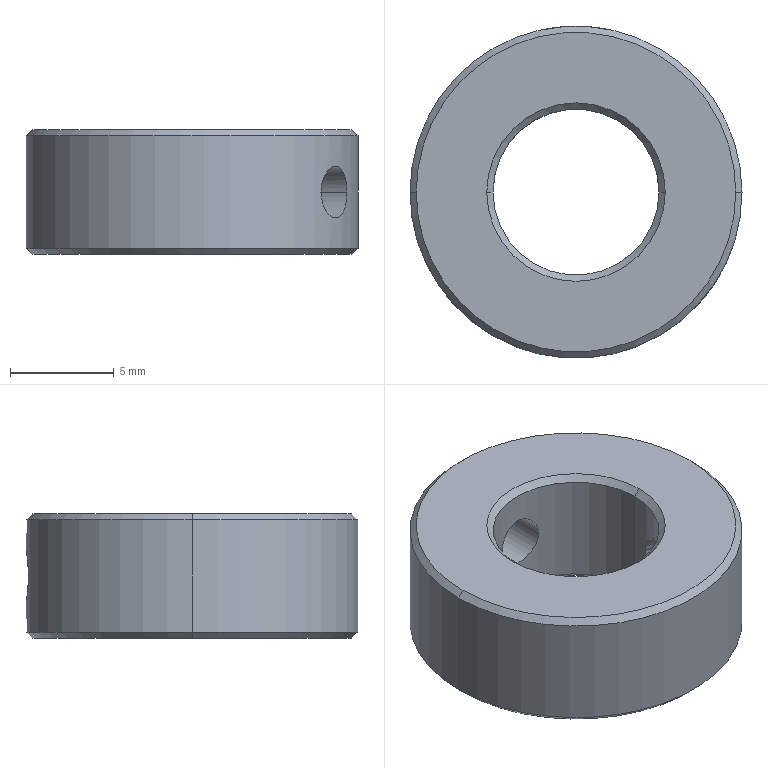Component | SolidWorks | LD101-02--Q1107-2-5 | 1 solid | 18 faces | box 16 x 16 x 6 mm | volume 858 mm3 | cylinder 8 | cone 8 | plane 2 | commonest cylinder face diameters 2.5 x4 8 x2 16 x2 | material 45
build123d program:
from build123d import *

# Parameters (mm, degrees)
SKETCH1_R           = 8
SKETCH1_R_2         = 4
BOSS_EXTRUDE1_DEPTH = 3
CHAMFER1_SIZE       = 0.3
SKETCH3_W           = 1.25
SKETCH3_H           = 8
CIRPATTERN1_COUNT   = 2
CIRPATTERN1_ANGLE   = 120


with BuildPart() as part:
    # Sketch1 → Boss-Extrude1 (new, symmetric)
    with BuildSketch(Plane.XY):
        Circle(SKETCH1_R)
        Circle(SKETCH1_R_2, mode=Mode.SUBTRACT)
    extrude(amount=BOSS_EXTRUDE1_DEPTH, both=True)

    # Chamfer1
    chamfer1_edges = [part.edges().sort_by_distance(p)[0] for p in [
        (-8, 0, -3),
        (-8, 0, 3),
        (-4, 0, -3),
        (-4, 0, 3),
    ]]
    chamfer(chamfer1_edges, length=CHAMFER1_SIZE)

    # Sketch3 → M3 Tapped Hole1 (revolve, cut)
    with BuildSketch(Plane(origin=(0, 0, 0), x_dir=(0, 0, -1), z_dir=(1, 0, 0))):
        with Locations((0.625, 4)):
            Rectangle(SKETCH3_W, SKETCH3_H)
    m3_tapped_hole1 = revolve(axis=Axis((0, -6.35, 0), (0, 1, 0)), mode=Mode.SUBTRACT)

    # CirPattern1: M3 Tapped Hole1 ×2 about axis
    cirpattern1_axis = Axis((0, 0, 3), (0, 0, -1))
    for i in range(1, CIRPATTERN1_COUNT):
        add(m3_tapped_hole1.rotate(cirpattern1_axis, i * CIRPATTERN1_ANGLE / (CIRPATTERN1_COUNT - 1)), mode=Mode.SUBTRACT)


solid = part.part

# Placed as in the assembly
solid = solid.moved(Location((79.71, -135.897, 296.257), (0, 0, 0)))
STEP:
#1=CARTESIAN_POINT('',(3.432,-5.463,11.664));
#2=VERTEX_POINT('',#1);
#3=CARTESIAN_POINT('',(3.383,-5.548,11.664));
#4=VERTEX_POINT('',#3);
#5=CARTESIAN_POINT('',(3.432,-5.463,11.664));
#6=CARTESIAN_POINT('',(3.432,-5.463,11.657));
#7=CARTESIAN_POINT('',(3.432,-5.464,11.651));
#8=CARTESIAN_POINT('',(3.43,-5.469,11.639));
#9=CARTESIAN_POINT('',(3.429,-5.472,11.633));
#10=CARTESIAN_POINT('',(3.426,-5.479,11.627));
#11=CARTESIAN_POINT('',(3.425,-5.481,11.625));
#12=CARTESIAN_POINT('',(3.422,-5.486,11.621));
#13=CARTESIAN_POINT('',(3.421,-5.488,11.619));
#14=CARTESIAN_POINT('',(3.417,-5.496,11.616));
#15=CARTESIAN_POINT('',(3.414,-5.502,11.614));
#16=CARTESIAN_POINT('',(3.408,-5.513,11.614));
#17=CARTESIAN_POINT('',(3.404,-5.519,11.616));
#18=CARTESIAN_POINT('',(3.398,-5.529,11.621));
#19=CARTESIAN_POINT('',(3.395,-5.533,11.624));
#20=CARTESIAN_POINT('',(3.389,-5.541,11.633));
#21=CARTESIAN_POINT('',(3.387,-5.544,11.639));
#22=CARTESIAN_POINT('',(3.384,-5.547,11.651));
#23=CARTESIAN_POINT('',(3.383,-5.548,11.657));
#24=CARTESIAN_POINT('',(3.383,-5.548,11.664));
#25=B_SPLINE_CURVE_WITH_KNOTS('',3,(#5,#6,#7,#8,#9,#10,#11,#12,#13,#14,#15,#16,#17,#18,#19,#20,#21,#22,#23,#24),.UNSPECIFIED.,.F.,.F.,(4,2,2,2,2,2,2,2,2,4),(0.003914,0.004403,0.004892,0.005137,0.005381,0.005871,0.00636,0.006849,0.007338,0.007827),.UNSPECIFIED.);
#26=EDGE_CURVE('',#2,#4,#25,.T.);
#27=ORIENTED_EDGE('',*,*,#26,.F.);
#28=CARTESIAN_POINT('',(3.292,-5.382,11.664));
#29=VERTEX_POINT('',#28);
#30=CARTESIAN_POINT('',(3.163,-5.308,11.664));
#31=DIRECTION('',(-0.866,0.5,0.));
#32=VECTOR('',#31,39.37);
#33=LINE('',#30,#32);
#34=EDGE_CURVE('',#2,#29,#33,.T.);
#35=ORIENTED_EDGE('',*,*,#34,.T.);
#36=CARTESIAN_POINT('',(3.243,-5.468,11.664));
#37=VERTEX_POINT('',#36);
#38=CARTESIAN_POINT('',(3.292,-5.382,11.664));
#39=CARTESIAN_POINT('',(3.292,-5.382,11.657));
#40=CARTESIAN_POINT('',(3.292,-5.384,11.651));
#41=CARTESIAN_POINT('',(3.291,-5.389,11.639));
#42=CARTESIAN_POINT('',(3.29,-5.392,11.633));
#43=CARTESIAN_POINT('',(3.287,-5.401,11.624));
#44=CARTESIAN_POINT('',(3.285,-5.407,11.621));
#45=CARTESIAN_POINT('',(3.282,-5.415,11.617));
#46=CARTESIAN_POINT('',(3.281,-5.418,11.616));
#47=CARTESIAN_POINT('',(3.278,-5.423,11.615));
#48=CARTESIAN_POINT('',(3.276,-5.426,11.614));
#49=CARTESIAN_POINT('',(3.271,-5.435,11.614));
#50=CARTESIAN_POINT('',(3.268,-5.44,11.616));
#51=CARTESIAN_POINT('',(3.261,-5.45,11.621));
#52=CARTESIAN_POINT('',(3.257,-5.454,11.624));
#53=CARTESIAN_POINT('',(3.251,-5.461,11.633));
#54=CARTESIAN_POINT('',(3.248,-5.463,11.639));
#55=CARTESIAN_POINT('',(3.244,-5.467,11.651));
#56=CARTESIAN_POINT('',(3.243,-5.468,11.657));
#57=CARTESIAN_POINT('',(3.243,-5.468,11.664));
#58=B_SPLINE_CURVE_WITH_KNOTS('',3,(#38,#39,#40,#41,#42,#43,#44,#45,#46,#47,#48,#49,#50,#51,#52,#53,#54,#55,#56,#57),.UNSPECIFIED.,.F.,.F.,(4,2,2,2,2,2,2,2,2,4),(0.003933,0.004424,0.004916,0.005407,0.005653,0.005899,0.00639,0.006882,0.007373,0.007864),.UNSPECIFIED.);
#59=EDGE_CURVE('',#29,#37,#58,.T.);
#60=ORIENTED_EDGE('',*,*,#59,.T.);
#61=CARTESIAN_POINT('',(3.114,-5.393,11.664));
#62=DIRECTION('',(-0.866,0.5,0.));
#63=VECTOR('',#62,39.37);
#64=LINE('',#61,#63);
#65=EDGE_CURVE('',#4,#37,#64,.T.);
#66=ORIENTED_EDGE('',*,*,#65,.F.);
#67=EDGE_LOOP('',(#27,#35,#60,#66));
#68=FACE_OUTER_BOUND('',#67,.T.);
#69=CARTESIAN_POINT('',(3.138,-5.35,11.664));
#70=DIRECTION('',(-0.866,0.5,0.));
#71=DIRECTION('',(-0.5,-0.866,0.));
#72=AXIS2_PLACEMENT_3D('',#69,#70,#71);
#73=CYLINDRICAL_SURFACE('',#72,0.04921);
#74=ADVANCED_FACE('',(#68),#73,.F.);
#75=CARTESIAN_POINT('',(3.138,-5.035,11.713));
#76=VERTEX_POINT('',#75);
#77=CARTESIAN_POINT('',(3.138,-5.035,11.614));
#78=VERTEX_POINT('',#77);
#79=CARTESIAN_POINT('',(3.138,-5.035,11.713));
#80=CARTESIAN_POINT('',(3.132,-5.035,11.713));
#81=CARTESIAN_POINT('',(3.125,-5.036,11.712));
#82=CARTESIAN_POINT('',(3.113,-5.036,11.707));
#83=CARTESIAN_POINT('',(3.108,-5.037,11.703));
#84=CARTESIAN_POINT('',(3.101,-5.037,11.696));
#85=CARTESIAN_POINT('',(3.099,-5.038,11.694));
#86=CARTESIAN_POINT('',(3.096,-5.038,11.688));
#87=CARTESIAN_POINT('',(3.094,-5.038,11.686));
#88=CARTESIAN_POINT('',(3.09,-5.039,11.677));
#89=CARTESIAN_POINT('',(3.089,-5.039,11.67));
#90=CARTESIAN_POINT('',(3.089,-5.039,11.657));
#91=CARTESIAN_POINT('',(3.09,-5.039,11.651));
#92=CARTESIAN_POINT('',(3.095,-5.038,11.639));
#93=CARTESIAN_POINT('',(3.099,-5.038,11.633));
#94=CARTESIAN_POINT('',(3.108,-5.037,11.624));
#95=CARTESIAN_POINT('',(3.113,-5.036,11.621));
#96=CARTESIAN_POINT('',(3.125,-5.036,11.616));
#97=CARTESIAN_POINT('',(3.132,-5.035,11.614));
#98=CARTESIAN_POINT('',(3.138,-5.035,11.614));
#99=B_SPLINE_CURVE_WITH_KNOTS('',3,(#79,#80,#81,#82,#83,#84,#85,#86,#87,#88,#89,#90,#91,#92,#93,#94,#95,#96,#97,#98),.UNSPECIFIED.,.F.,.F.,(4,2,2,2,2,2,2,2,2,4),(0.003914,0.004403,0.004892,0.005137,0.005381,0.005871,0.00636,0.006849,0.007338,0.007827),.UNSPECIFIED.);
#100=EDGE_CURVE('',#76,#78,#99,.T.);
#101=ORIENTED_EDGE('',*,*,#100,.F.);
#102=CARTESIAN_POINT('',(3.138,-5.193,11.713));
#103=VERTEX_POINT('',#102);
#104=CARTESIAN_POINT('',(3.138,-5.35,11.713));
#105=DIRECTION('',(0.,-1.,0.));
#106=VECTOR('',#105,39.37);
#107=LINE('',#104,#106);
#108=EDGE_CURVE('',#76,#103,#107,.T.);
#109=ORIENTED_EDGE('',*,*,#108,.T.);
#110=CARTESIAN_POINT('',(3.138,-5.193,11.614));
#111=VERTEX_POINT('',#110);
#112=CARTESIAN_POINT('',(3.138,-5.193,11.713));
#113=CARTESIAN_POINT('',(3.132,-5.193,11.713));
#114=CARTESIAN_POINT('',(3.125,-5.193,11.712));
#115=CARTESIAN_POINT('',(3.113,-5.195,11.707));
#116=CARTESIAN_POINT('',(3.108,-5.196,11.703));
#117=CARTESIAN_POINT('',(3.099,-5.198,11.694));
#118=CARTESIAN_POINT('',(3.095,-5.199,11.689));
#119=CARTESIAN_POINT('',(3.092,-5.2,11.68));
#120=CARTESIAN_POINT('',(3.091,-5.2,11.676));
#121=CARTESIAN_POINT('',(3.089,-5.201,11.67));
#122=CARTESIAN_POINT('',(3.089,-5.201,11.667));
#123=CARTESIAN_POINT('',(3.089,-5.201,11.657));
#124=CARTESIAN_POINT('',(3.09,-5.2,11.651));
#125=CARTESIAN_POINT('',(3.095,-5.199,11.639));
#126=CARTESIAN_POINT('',(3.099,-5.198,11.633));
#127=CARTESIAN_POINT('',(3.108,-5.196,11.624));
#128=CARTESIAN_POINT('',(3.113,-5.195,11.621));
#129=CARTESIAN_POINT('',(3.125,-5.193,11.616));
#130=CARTESIAN_POINT('',(3.132,-5.193,11.614));
#131=CARTESIAN_POINT('',(3.138,-5.193,11.614));
#132=B_SPLINE_CURVE_WITH_KNOTS('',3,(#112,#113,#114,#115,#116,#117,#118,#119,#120,#121,#122,#123,#124,#125,#126,#127,#128,#129,#130,#131),.UNSPECIFIED.,.F.,.F.,(4,2,2,2,2,2,2,2,2,4),(0.003933,0.004424,0.004916,0.005407,0.005653,0.005899,0.00639,0.006882,0.007373,0.007865),.UNSPECIFIED.);
#133=EDGE_CURVE('',#103,#111,#132,.T.);
#134=ORIENTED_EDGE('',*,*,#133,.T.);
#135=CARTESIAN_POINT('',(3.138,-5.35,11.614));
#136=DIRECTION('',(0.,-1.,0.));
#137=VECTOR('',#136,39.37);
#138=LINE('',#135,#137);
#139=EDGE_CURVE('',#78,#111,#138,.T.);
#140=ORIENTED_EDGE('',*,*,#139,.F.);
#141=EDGE_LOOP('',(#101,#109,#134,#140));
#142=FACE_OUTER_BOUND('',#141,.T.);
#143=CARTESIAN_POINT('',(3.138,-5.35,11.664));
#144=DIRECTION('',(0.,-1.,0.));
#145=DIRECTION('',(0.,0.,-1.));
#146=AXIS2_PLACEMENT_3D('',#143,#144,#145);
#147=CYLINDRICAL_SURFACE('',#146,0.04921);
#148=ADVANCED_FACE('',(#142),#147,.F.);
#149=CARTESIAN_POINT('',(3.441,-5.35,11.782));
#150=VERTEX_POINT('',#149);
#151=CARTESIAN_POINT('',(2.835,-5.35,11.782));
#152=VERTEX_POINT('',#151);
#153=CARTESIAN_POINT('',(3.138,-5.35,11.782));
#154=DIRECTION('',(0.,0.,1.));
#155=DIRECTION('',(1.,0.,0.));
#156=AXIS2_PLACEMENT_3D('',#153,#154,#155);
#157=CIRCLE('',#156,0.3031);
#158=EDGE_CURVE('',#150,#152,#157,.T.);
#159=ORIENTED_EDGE('',*,*,#158,.F.);
#160=CARTESIAN_POINT('',(3.453,-5.35,11.77));
#161=VERTEX_POINT('',#160);
#162=CARTESIAN_POINT('',(3.441,-5.35,11.782));
#163=DIRECTION('',(0.7071,0.,-0.7071));
#164=VECTOR('',#163,39.37);
#165=LINE('',#162,#164);
#166=EDGE_CURVE('',#150,#161,#165,.T.);
#167=ORIENTED_EDGE('',*,*,#166,.T.);
#168=CARTESIAN_POINT('',(2.823,-5.35,11.77));
#169=VERTEX_POINT('',#168);
#170=CARTESIAN_POINT('',(3.138,-5.35,11.77));
#171=DIRECTION('',(0.,0.,-1.));
#172=DIRECTION('',(1.,0.,0.));
#173=AXIS2_PLACEMENT_3D('',#170,#171,#172);
#174=CIRCLE('',#173,0.315);
#175=EDGE_CURVE('',#169,#161,#174,.T.);
#176=ORIENTED_EDGE('',*,*,#175,.F.);
#177=CARTESIAN_POINT('',(2.835,-5.35,11.782));
#178=DIRECTION('',(-0.7071,0.,-0.7071));
#179=VECTOR('',#178,39.37);
#180=LINE('',#177,#179);
#181=EDGE_CURVE('',#152,#169,#180,.T.);
#182=ORIENTED_EDGE('',*,*,#181,.F.);
#183=EDGE_LOOP('',(#159,#167,#176,#182));
#184=FACE_OUTER_BOUND('',#183,.T.);
#185=CARTESIAN_POINT('',(3.138,-5.35,11.782));
#186=DIRECTION('',(0.,0.,-1.));
#187=DIRECTION('',(-1.,0.,0.));
#188=AXIS2_PLACEMENT_3D('',#185,#186,#187);
#189=CONICAL_SURFACE('',#188,0.3031,0.7854);
#190=ADVANCED_FACE('',(#184),#189,.T.);
#191=CARTESIAN_POINT('',(2.981,-5.35,11.77));
#192=VERTEX_POINT('',#191);
#193=CARTESIAN_POINT('',(3.296,-5.35,11.77));
#194=VERTEX_POINT('',#193);
#195=CARTESIAN_POINT('',(3.138,-5.35,11.77));
#196=DIRECTION('',(0.,0.,1.));
#197=DIRECTION('',(1.,0.,0.));
#198=AXIS2_PLACEMENT_3D('',#195,#196,#197);
#199=CIRCLE('',#198,0.1575);
#200=EDGE_CURVE('',#192,#194,#199,.T.);
#201=ORIENTED_EDGE('',*,*,#200,.F.);
#202=CARTESIAN_POINT('',(2.969,-5.35,11.782));
#203=VERTEX_POINT('',#202);
#204=CARTESIAN_POINT('',(2.981,-5.35,11.77));
#205=DIRECTION('',(-0.7071,0.,0.7071));
#206=VECTOR('',#205,39.37);
#207=LINE('',#204,#206);
#208=EDGE_CURVE('',#192,#203,#207,.T.);
#209=ORIENTED_EDGE('',*,*,#208,.T.);
#210=CARTESIAN_POINT('',(3.307,-5.35,11.782));
#211=VERTEX_POINT('',#210);
#212=CARTESIAN_POINT('',(3.138,-5.35,11.782));
#213=DIRECTION('',(0.,0.,-1.));
#214=DIRECTION('',(1.,0.,0.));
#215=AXIS2_PLACEMENT_3D('',#212,#213,#214);
#216=CIRCLE('',#215,0.1693);
#217=EDGE_CURVE('',#211,#203,#216,.T.);
#218=ORIENTED_EDGE('',*,*,#217,.F.);
#219=CARTESIAN_POINT('',(3.296,-5.35,11.77));
#220=DIRECTION('',(0.7071,0.,0.7071));
#221=VECTOR('',#220,39.37);
#222=LINE('',#219,#221);
#223=EDGE_CURVE('',#194,#211,#222,.T.);
#224=ORIENTED_EDGE('',*,*,#223,.F.);
#225=EDGE_LOOP('',(#201,#209,#218,#224));
#226=FACE_OUTER_BOUND('',#225,.T.);
#227=CARTESIAN_POINT('',(3.138,-5.35,11.77));
#228=DIRECTION('',(0.,0.,1.));
#229=DIRECTION('',(1.,0.,0.));
#230=AXIS2_PLACEMENT_3D('',#227,#228,#229);
#231=CONICAL_SURFACE('',#230,0.1575,0.7854);
#232=ADVANCED_FACE('',(#226),#231,.F.);
#233=CARTESIAN_POINT('',(2.835,-5.35,11.546));
#234=VERTEX_POINT('',#233);
#235=CARTESIAN_POINT('',(3.441,-5.35,11.546));
#236=VERTEX_POINT('',#235);
#237=CARTESIAN_POINT('',(3.138,-5.35,11.546));
#238=DIRECTION('',(0.,0.,-1.));
#239=DIRECTION('',(1.,0.,0.));
#240=AXIS2_PLACEMENT_3D('',#237,#238,#239);
#241=CIRCLE('',#240,0.3031);
#242=EDGE_CURVE('',#234,#236,#241,.T.);
#243=ORIENTED_EDGE('',*,*,#242,.F.);
#244=CARTESIAN_POINT('',(2.823,-5.35,11.557));
#245=VERTEX_POINT('',#244);
#246=CARTESIAN_POINT('',(2.823,-5.35,11.557));
#247=DIRECTION('',(-0.7071,0.,0.7071));
#248=VECTOR('',#247,39.37);
#249=LINE('',#246,#248);
#250=EDGE_CURVE('',#234,#245,#249,.T.);
#251=ORIENTED_EDGE('',*,*,#250,.T.);
#252=CARTESIAN_POINT('',(3.453,-5.35,11.557));
#253=VERTEX_POINT('',#252);
#254=CARTESIAN_POINT('',(3.138,-5.35,11.557));
#255=DIRECTION('',(0.,0.,1.));
#256=DIRECTION('',(1.,0.,0.));
#257=AXIS2_PLACEMENT_3D('',#254,#255,#256);
#258=CIRCLE('',#257,0.315);
#259=EDGE_CURVE('',#253,#245,#258,.T.);
#260=ORIENTED_EDGE('',*,*,#259,.F.);
#261=CARTESIAN_POINT('',(3.453,-5.35,11.557));
#262=DIRECTION('',(0.7071,0.,0.7071));
#263=VECTOR('',#262,39.37);
#264=LINE('',#261,#263);
#265=EDGE_CURVE('',#236,#253,#264,.T.);
#266=ORIENTED_EDGE('',*,*,#265,.F.);
#267=EDGE_LOOP('',(#243,#251,#260,#266));
#268=FACE_OUTER_BOUND('',#267,.T.);
#269=CARTESIAN_POINT('',(3.138,-5.35,11.557));
#270=DIRECTION('',(0.,0.,1.));
#271=DIRECTION('',(1.,0.,0.));
#272=AXIS2_PLACEMENT_3D('',#269,#270,#271);
#273=CONICAL_SURFACE('',#272,0.315,0.7854);
#274=ADVANCED_FACE('',(#268),#273,.T.);
#275=CARTESIAN_POINT('',(3.296,-5.35,11.557));
#276=VERTEX_POINT('',#275);
#277=CARTESIAN_POINT('',(2.981,-5.35,11.557));
#278=VERTEX_POINT('',#277);
#279=CARTESIAN_POINT('',(3.138,-5.35,11.557));
#280=DIRECTION('',(0.,0.,-1.));
#281=DIRECTION('',(1.,0.,0.));
#282=AXIS2_PLACEMENT_3D('',#279,#280,#281);
#283=CIRCLE('',#282,0.1575);
#284=EDGE_CURVE('',#276,#278,#283,.T.);
#285=ORIENTED_EDGE('',*,*,#284,.F.);
#286=CARTESIAN_POINT('',(3.307,-5.35,11.546));
#287=VERTEX_POINT('',#286);
#288=CARTESIAN_POINT('',(3.307,-5.35,11.546));
#289=DIRECTION('',(0.7071,0.,-0.7071));
#290=VECTOR('',#289,39.37);
#291=LINE('',#288,#290);
#292=EDGE_CURVE('',#276,#287,#291,.T.);
#293=ORIENTED_EDGE('',*,*,#292,.T.);
#294=CARTESIAN_POINT('',(2.969,-5.35,11.546));
#295=VERTEX_POINT('',#294);
#296=CARTESIAN_POINT('',(3.138,-5.35,11.546));
#297=DIRECTION('',(0.,0.,1.));
#298=DIRECTION('',(1.,0.,0.));
#299=AXIS2_PLACEMENT_3D('',#296,#297,#298);
#300=CIRCLE('',#299,0.1693);
#301=EDGE_CURVE('',#295,#287,#300,.T.);
#302=ORIENTED_EDGE('',*,*,#301,.F.);
#303=CARTESIAN_POINT('',(2.969,-5.35,11.546));
#304=DIRECTION('',(-0.7071,0.,-0.7071));
#305=VECTOR('',#304,39.37);
#306=LINE('',#303,#305);
#307=EDGE_CURVE('',#278,#295,#306,.T.);
#308=ORIENTED_EDGE('',*,*,#307,.F.);
#309=EDGE_LOOP('',(#285,#293,#302,#308));
#310=FACE_OUTER_BOUND('',#309,.T.);
#311=CARTESIAN_POINT('',(3.138,-5.35,11.546));
#312=DIRECTION('',(0.,0.,-1.));
#313=DIRECTION('',(-1.,0.,0.));
#314=AXIS2_PLACEMENT_3D('',#311,#312,#313);
#315=CONICAL_SURFACE('',#314,0.1693,0.7854);
#316=ADVANCED_FACE('',(#310),#315,.F.);
#317=CARTESIAN_POINT('',(3.243,-5.468,11.664));
#318=CARTESIAN_POINT('',(3.243,-5.468,11.67));
#319=CARTESIAN_POINT('',(3.244,-5.467,11.677));
#320=CARTESIAN_POINT('',(3.248,-5.463,11.689));
#321=CARTESIAN_POINT('',(3.251,-5.461,11.694));
#322=CARTESIAN_POINT('',(3.257,-5.454,11.703));
#323=CARTESIAN_POINT('',(3.261,-5.45,11.707));
#324=CARTESIAN_POINT('',(3.268,-5.44,11.712));
#325=CARTESIAN_POINT('',(3.271,-5.435,11.713));
#326=CARTESIAN_POINT('',(3.276,-5.426,11.713));
#327=CARTESIAN_POINT('',(3.278,-5.423,11.713));
#328=CARTESIAN_POINT('',(3.281,-5.418,11.711));
#329=CARTESIAN_POINT('',(3.282,-5.415,11.71));
#330=CARTESIAN_POINT('',(3.285,-5.407,11.707));
#331=CARTESIAN_POINT('',(3.287,-5.401,11.703));
#332=CARTESIAN_POINT('',(3.289,-5.395,11.696));
#333=CARTESIAN_POINT('',(3.29,-5.393,11.694));
#334=CARTESIAN_POINT('',(3.291,-5.389,11.688));
#335=CARTESIAN_POINT('',(3.291,-5.388,11.685));
#336=CARTESIAN_POINT('',(3.292,-5.384,11.677));
#337=CARTESIAN_POINT('',(3.292,-5.382,11.67));
#338=CARTESIAN_POINT('',(3.292,-5.382,11.664));
#339=B_SPLINE_CURVE_WITH_KNOTS('',3,(#317,#318,#319,#320,#321,#322,#323,#324,#325,#326,#327,#328,#329,#330,#331,#332,#333,#334,#335,#336,#337,#338),.UNSPECIFIED.,.F.,.F.,(4,2,2,2,2,2,2,2,2,2,4),(0.,0.0004916,0.0009832,0.001475,0.001966,0.002212,0.002458,0.00295,0.003195,0.003441,0.003933),.UNSPECIFIED.);
#340=EDGE_CURVE('',#37,#29,#339,.T.);
#341=ORIENTED_EDGE('',*,*,#340,.F.);
#342=ORIENTED_EDGE('',*,*,#59,.F.);
#343=EDGE_LOOP('',(#341,#342));
#344=FACE_BOUND('',#343,.T.);
#345=ORIENTED_EDGE('',*,*,#200,.T.);
#346=CARTESIAN_POINT('',(3.296,-5.35,11.782));
#347=DIRECTION('',(0.,0.,-1.));
#348=VECTOR('',#347,39.37);
#349=LINE('',#346,#348);
#350=EDGE_CURVE('',#194,#276,#349,.T.);
#351=ORIENTED_EDGE('',*,*,#350,.T.);
#352=ORIENTED_EDGE('',*,*,#284,.T.);
#353=CARTESIAN_POINT('',(2.981,-5.35,11.782));
#354=DIRECTION('',(0.,0.,-1.));
#355=VECTOR('',#354,39.37);
#356=LINE('',#353,#355);
#357=EDGE_CURVE('',#192,#278,#356,.T.);
#358=ORIENTED_EDGE('',*,*,#357,.F.);
#359=EDGE_LOOP('',(#345,#351,#352,#358));
#360=FACE_OUTER_BOUND('',#359,.T.);
#361=CARTESIAN_POINT('',(3.138,-5.35,11.782));
#362=DIRECTION('',(0.,0.,-1.));
#363=DIRECTION('',(-1.,0.,0.));
#364=AXIS2_PLACEMENT_3D('',#361,#362,#363);
#365=CYLINDRICAL_SURFACE('',#364,0.1575);
#366=ADVANCED_FACE('',(#344,#360),#365,.F.);
#367=CARTESIAN_POINT('',(3.138,-5.035,11.614));
#368=CARTESIAN_POINT('',(3.145,-5.035,11.614));
#369=CARTESIAN_POINT('',(3.151,-5.036,11.616));
#370=CARTESIAN_POINT('',(3.163,-5.036,11.621));
#371=CARTESIAN_POINT('',(3.168,-5.037,11.624));
#372=CARTESIAN_POINT('',(3.178,-5.038,11.633));
#373=CARTESIAN_POINT('',(3.181,-5.038,11.639));
#374=CARTESIAN_POINT('',(3.186,-5.039,11.651));
#375=CARTESIAN_POINT('',(3.187,-5.039,11.657));
#376=CARTESIAN_POINT('',(3.187,-5.039,11.667));
#377=CARTESIAN_POINT('',(3.187,-5.039,11.67));
#378=CARTESIAN_POINT('',(3.186,-5.039,11.676));
#379=CARTESIAN_POINT('',(3.185,-5.039,11.679));
#380=CARTESIAN_POINT('',(3.181,-5.038,11.688));
#381=CARTESIAN_POINT('',(3.178,-5.038,11.694));
#382=CARTESIAN_POINT('',(3.168,-5.037,11.703));
#383=CARTESIAN_POINT('',(3.163,-5.036,11.707));
#384=CARTESIAN_POINT('',(3.154,-5.036,11.71));
#385=CARTESIAN_POINT('',(3.151,-5.036,11.711));
#386=CARTESIAN_POINT('',(3.145,-5.035,11.713));
#387=CARTESIAN_POINT('',(3.141,-5.035,11.713));
#388=CARTESIAN_POINT('',(3.138,-5.035,11.713));
#389=B_SPLINE_CURVE_WITH_KNOTS('',3,(#367,#368,#369,#370,#371,#372,#373,#374,#375,#376,#377,#378,#379,#380,#381,#382,#383,#384,#385,#386,#387,#388),.UNSPECIFIED.,.F.,.F.,(4,2,2,2,2,2,2,2,2,2,4),(0.,0.0004893,0.0009785,0.001468,0.001957,0.002202,0.002446,0.002936,0.003425,0.003669,0.003914),.UNSPECIFIED.);
#390=EDGE_CURVE('',#78,#76,#389,.T.);
#391=ORIENTED_EDGE('',*,*,#390,.T.);
#392=ORIENTED_EDGE('',*,*,#100,.T.);
#393=EDGE_LOOP('',(#391,#392));
#394=FACE_BOUND('',#393,.T.);
#395=ORIENTED_EDGE('',*,*,#175,.T.);
#396=CARTESIAN_POINT('',(3.453,-5.35,11.782));
#397=DIRECTION('',(0.,0.,-1.));
#398=VECTOR('',#397,39.37);
#399=LINE('',#396,#398);
#400=EDGE_CURVE('',#161,#253,#399,.T.);
#401=ORIENTED_EDGE('',*,*,#400,.T.);
#402=ORIENTED_EDGE('',*,*,#259,.T.);
#403=CARTESIAN_POINT('',(2.823,-5.35,11.782));
#404=DIRECTION('',(0.,0.,-1.));
#405=VECTOR('',#404,39.37);
#406=LINE('',#403,#405);
#407=EDGE_CURVE('',#169,#245,#406,.T.);
#408=ORIENTED_EDGE('',*,*,#407,.F.);
#409=EDGE_LOOP('',(#395,#401,#402,#408));
#410=FACE_OUTER_BOUND('',#409,.T.);
#411=CARTESIAN_POINT('',(3.138,-5.35,11.782));
#412=DIRECTION('',(0.,0.,-1.));
#413=DIRECTION('',(-1.,0.,0.));
#414=AXIS2_PLACEMENT_3D('',#411,#412,#413);
#415=CYLINDRICAL_SURFACE('',#414,0.315);
#416=ADVANCED_FACE('',(#394,#410),#415,.T.);
#417=ORIENTED_EDGE('',*,*,#217,.T.);
#418=CARTESIAN_POINT('',(3.138,-5.35,11.782));
#419=DIRECTION('',(0.,0.,-1.));
#420=DIRECTION('',(1.,0.,0.));
#421=AXIS2_PLACEMENT_3D('',#418,#419,#420);
#422=CIRCLE('',#421,0.1693);
#423=EDGE_CURVE('',#203,#211,#422,.T.);
#424=ORIENTED_EDGE('',*,*,#423,.T.);
#425=EDGE_LOOP('',(#417,#424));
#426=FACE_BOUND('',#425,.T.);
#427=CARTESIAN_POINT('',(3.138,-5.35,11.782));
#428=DIRECTION('',(0.,0.,1.));
#429=DIRECTION('',(1.,0.,0.));
#430=AXIS2_PLACEMENT_3D('',#427,#428,#429);
#431=CIRCLE('',#430,0.3031);
#432=EDGE_CURVE('',#152,#150,#431,.T.);
#433=ORIENTED_EDGE('',*,*,#432,.T.);
#434=ORIENTED_EDGE('',*,*,#158,.T.);
#435=EDGE_LOOP('',(#433,#434));
#436=FACE_OUTER_BOUND('',#435,.T.);
#437=CARTESIAN_POINT('',(3.138,-5.35,11.782));
#438=DIRECTION('',(0.,0.,1.));
#439=DIRECTION('',(1.,0.,0.));
#440=AXIS2_PLACEMENT_3D('',#437,#438,#439);
#441=PLANE('',#440);
#442=ADVANCED_FACE('',(#426,#436),#441,.T.);
#443=ORIENTED_EDGE('',*,*,#301,.T.);
#444=CARTESIAN_POINT('',(3.138,-5.35,11.546));
#445=DIRECTION('',(0.,0.,1.));
#446=DIRECTION('',(1.,0.,0.));
#447=AXIS2_PLACEMENT_3D('',#444,#445,#446);
#448=CIRCLE('',#447,0.1693);
#449=EDGE_CURVE('',#287,#295,#448,.T.);
#450=ORIENTED_EDGE('',*,*,#449,.T.);
#451=EDGE_LOOP('',(#443,#450));
#452=FACE_BOUND('',#451,.T.);
#453=CARTESIAN_POINT('',(3.138,-5.35,11.546));
#454=DIRECTION('',(0.,0.,-1.));
#455=DIRECTION('',(1.,0.,0.));
#456=AXIS2_PLACEMENT_3D('',#453,#454,#455);
#457=CIRCLE('',#456,0.3031);
#458=EDGE_CURVE('',#236,#234,#457,.T.);
#459=ORIENTED_EDGE('',*,*,#458,.T.);
#460=ORIENTED_EDGE('',*,*,#242,.T.);
#461=EDGE_LOOP('',(#459,#460));
#462=FACE_OUTER_BOUND('',#461,.T.);
#463=CARTESIAN_POINT('',(3.138,-5.35,11.546));
#464=DIRECTION('',(0.,0.,1.));
#465=DIRECTION('',(1.,0.,0.));
#466=AXIS2_PLACEMENT_3D('',#463,#464,#465);
#467=PLANE('',#466);
#468=ADVANCED_FACE('',(#452,#462),#467,.F.);
#469=ORIENTED_EDGE('',*,*,#400,.F.);
#470=CARTESIAN_POINT('',(3.138,-5.35,11.77));
#471=DIRECTION('',(0.,0.,-1.));
#472=DIRECTION('',(1.,0.,0.));
#473=AXIS2_PLACEMENT_3D('',#470,#471,#472);
#474=CIRCLE('',#473,0.315);
#475=EDGE_CURVE('',#161,#169,#474,.T.);
#476=ORIENTED_EDGE('',*,*,#475,.T.);
#477=ORIENTED_EDGE('',*,*,#407,.T.);
#478=CARTESIAN_POINT('',(3.138,-5.35,11.557));
#479=DIRECTION('',(0.,0.,1.));
#480=DIRECTION('',(1.,0.,0.));
#481=AXIS2_PLACEMENT_3D('',#478,#479,#480);
#482=CIRCLE('',#481,0.315);
#483=EDGE_CURVE('',#245,#253,#482,.T.);
#484=ORIENTED_EDGE('',*,*,#483,.T.);
#485=EDGE_LOOP('',(#469,#476,#477,#484));
#486=FACE_OUTER_BOUND('',#485,.T.);
#487=CARTESIAN_POINT('',(3.383,-5.548,11.664));
#488=CARTESIAN_POINT('',(3.383,-5.548,11.67));
#489=CARTESIAN_POINT('',(3.384,-5.547,11.677));
#490=CARTESIAN_POINT('',(3.387,-5.544,11.688));
#491=CARTESIAN_POINT('',(3.389,-5.541,11.694));
#492=CARTESIAN_POINT('',(3.395,-5.533,11.703));
#493=CARTESIAN_POINT('',(3.398,-5.529,11.707));
#494=CARTESIAN_POINT('',(3.404,-5.519,11.712));
#495=CARTESIAN_POINT('',(3.408,-5.513,11.713));
#496=CARTESIAN_POINT('',(3.413,-5.505,11.713));
#497=CARTESIAN_POINT('',(3.414,-5.502,11.713));
#498=CARTESIAN_POINT('',(3.417,-5.497,11.711));
#499=CARTESIAN_POINT('',(3.419,-5.494,11.71));
#500=CARTESIAN_POINT('',(3.423,-5.486,11.707));
#501=CARTESIAN_POINT('',(3.425,-5.481,11.703));
#502=CARTESIAN_POINT('',(3.429,-5.472,11.694));
#503=CARTESIAN_POINT('',(3.43,-5.469,11.688));
#504=CARTESIAN_POINT('',(3.431,-5.466,11.68));
#505=CARTESIAN_POINT('',(3.432,-5.465,11.676));
#506=CARTESIAN_POINT('',(3.432,-5.464,11.67));
#507=CARTESIAN_POINT('',(3.432,-5.463,11.667));
#508=CARTESIAN_POINT('',(3.432,-5.463,11.664));
#509=B_SPLINE_CURVE_WITH_KNOTS('',3,(#487,#488,#489,#490,#491,#492,#493,#494,#495,#496,#497,#498,#499,#500,#501,#502,#503,#504,#505,#506,#507,#508),.UNSPECIFIED.,.F.,.F.,(4,2,2,2,2,2,2,2,2,2,4),(0.,0.0004893,0.0009785,0.001468,0.001957,0.002202,0.002446,0.002936,0.003425,0.003669,0.003914),.UNSPECIFIED.);
#510=EDGE_CURVE('',#4,#2,#509,.T.);
#511=ORIENTED_EDGE('',*,*,#510,.T.);
#512=ORIENTED_EDGE('',*,*,#26,.T.);
#513=EDGE_LOOP('',(#511,#512));
#514=FACE_BOUND('',#513,.T.);
#515=CARTESIAN_POINT('',(3.138,-5.35,11.782));
#516=DIRECTION('',(0.,0.,-1.));
#517=DIRECTION('',(-1.,0.,0.));
#518=AXIS2_PLACEMENT_3D('',#515,#516,#517);
#519=CYLINDRICAL_SURFACE('',#518,0.315);
#520=ADVANCED_FACE('',(#486,#514),#519,.T.);
#521=ORIENTED_EDGE('',*,*,#350,.F.);
#522=CARTESIAN_POINT('',(3.138,-5.35,11.77));
#523=DIRECTION('',(0.,0.,1.));
#524=DIRECTION('',(1.,0.,0.));
#525=AXIS2_PLACEMENT_3D('',#522,#523,#524);
#526=CIRCLE('',#525,0.1575);
#527=EDGE_CURVE('',#194,#192,#526,.T.);
#528=ORIENTED_EDGE('',*,*,#527,.T.);
#529=ORIENTED_EDGE('',*,*,#357,.T.);
#530=CARTESIAN_POINT('',(3.138,-5.35,11.557));
#531=DIRECTION('',(0.,0.,-1.));
#532=DIRECTION('',(1.,0.,0.));
#533=AXIS2_PLACEMENT_3D('',#530,#531,#532);
#534=CIRCLE('',#533,0.1575);
#535=EDGE_CURVE('',#278,#276,#534,.T.);
#536=ORIENTED_EDGE('',*,*,#535,.T.);
#537=EDGE_LOOP('',(#521,#528,#529,#536));
#538=FACE_OUTER_BOUND('',#537,.T.);
#539=CARTESIAN_POINT('',(3.138,-5.193,11.614));
#540=CARTESIAN_POINT('',(3.145,-5.193,11.614));
#541=CARTESIAN_POINT('',(3.151,-5.193,11.616));
#542=CARTESIAN_POINT('',(3.163,-5.195,11.621));
#543=CARTESIAN_POINT('',(3.169,-5.196,11.624));
#544=CARTESIAN_POINT('',(3.178,-5.198,11.633));
#545=CARTESIAN_POINT('',(3.181,-5.199,11.639));
#546=CARTESIAN_POINT('',(3.186,-5.2,11.651));
#547=CARTESIAN_POINT('',(3.187,-5.201,11.657));
#548=CARTESIAN_POINT('',(3.187,-5.201,11.667));
#549=CARTESIAN_POINT('',(3.187,-5.201,11.67));
#550=CARTESIAN_POINT('',(3.186,-5.2,11.676));
#551=CARTESIAN_POINT('',(3.185,-5.2,11.68));
#552=CARTESIAN_POINT('',(3.181,-5.199,11.689));
#553=CARTESIAN_POINT('',(3.178,-5.198,11.694));
#554=CARTESIAN_POINT('',(3.171,-5.196,11.701));
#555=CARTESIAN_POINT('',(3.168,-5.196,11.703));
#556=CARTESIAN_POINT('',(3.163,-5.195,11.706));
#557=CARTESIAN_POINT('',(3.16,-5.194,11.708));
#558=CARTESIAN_POINT('',(3.151,-5.193,11.712));
#559=CARTESIAN_POINT('',(3.145,-5.193,11.713));
#560=CARTESIAN_POINT('',(3.138,-5.193,11.713));
#561=B_SPLINE_CURVE_WITH_KNOTS('',3,(#539,#540,#541,#542,#543,#544,#545,#546,#547,#548,#549,#550,#551,#552,#553,#554,#555,#556,#557,#558,#559,#560),.UNSPECIFIED.,.F.,.F.,(4,2,2,2,2,2,2,2,2,2,4),(0.,0.0004916,0.0009832,0.001475,0.001966,0.002212,0.002458,0.00295,0.003195,0.003441,0.003933),.UNSPECIFIED.);
#562=EDGE_CURVE('',#111,#103,#561,.T.);
#563=ORIENTED_EDGE('',*,*,#562,.F.);
#564=ORIENTED_EDGE('',*,*,#133,.F.);
#565=EDGE_LOOP('',(#563,#564));
#566=FACE_BOUND('',#565,.T.);
#567=CARTESIAN_POINT('',(3.138,-5.35,11.782));
#568=DIRECTION('',(0.,0.,-1.));
#569=DIRECTION('',(-1.,0.,0.));
#570=AXIS2_PLACEMENT_3D('',#567,#568,#569);
#571=CYLINDRICAL_SURFACE('',#570,0.1575);
#572=ADVANCED_FACE('',(#538,#566),#571,.F.);
#573=ORIENTED_EDGE('',*,*,#292,.F.);
#574=ORIENTED_EDGE('',*,*,#535,.F.);
#575=ORIENTED_EDGE('',*,*,#307,.T.);
#576=ORIENTED_EDGE('',*,*,#449,.F.);
#577=EDGE_LOOP('',(#573,#574,#575,#576));
#578=FACE_OUTER_BOUND('',#577,.T.);
#579=CARTESIAN_POINT('',(3.138,-5.35,11.546));
#580=DIRECTION('',(0.,0.,-1.));
#581=DIRECTION('',(-1.,0.,0.));
#582=AXIS2_PLACEMENT_3D('',#579,#580,#581);
#583=CONICAL_SURFACE('',#582,0.1693,0.7854);
#584=ADVANCED_FACE('',(#578),#583,.F.);
#585=ORIENTED_EDGE('',*,*,#250,.F.);
#586=ORIENTED_EDGE('',*,*,#458,.F.);
#587=ORIENTED_EDGE('',*,*,#265,.T.);
#588=ORIENTED_EDGE('',*,*,#483,.F.);
#589=EDGE_LOOP('',(#585,#586,#587,#588));
#590=FACE_OUTER_BOUND('',#589,.T.);
#591=CARTESIAN_POINT('',(3.138,-5.35,11.557));
#592=DIRECTION('',(0.,0.,1.));
#593=DIRECTION('',(1.,0.,0.));
#594=AXIS2_PLACEMENT_3D('',#591,#592,#593);
#595=CONICAL_SURFACE('',#594,0.315,0.7854);
#596=ADVANCED_FACE('',(#590),#595,.T.);
#597=ORIENTED_EDGE('',*,*,#208,.F.);
#598=ORIENTED_EDGE('',*,*,#527,.F.);
#599=ORIENTED_EDGE('',*,*,#223,.T.);
#600=ORIENTED_EDGE('',*,*,#423,.F.);
#601=EDGE_LOOP('',(#597,#598,#599,#600));
#602=FACE_OUTER_BOUND('',#601,.T.);
#603=CARTESIAN_POINT('',(3.138,-5.35,11.77));
#604=DIRECTION('',(0.,0.,1.));
#605=DIRECTION('',(1.,0.,0.));
#606=AXIS2_PLACEMENT_3D('',#603,#604,#605);
#607=CONICAL_SURFACE('',#606,0.1575,0.7854);
#608=ADVANCED_FACE('',(#602),#607,.F.);
#609=ORIENTED_EDGE('',*,*,#166,.F.);
#610=ORIENTED_EDGE('',*,*,#432,.F.);
#611=ORIENTED_EDGE('',*,*,#181,.T.);
#612=ORIENTED_EDGE('',*,*,#475,.F.);
#613=EDGE_LOOP('',(#609,#610,#611,#612));
#614=FACE_OUTER_BOUND('',#613,.T.);
#615=CARTESIAN_POINT('',(3.138,-5.35,11.782));
#616=DIRECTION('',(0.,0.,-1.));
#617=DIRECTION('',(-1.,0.,0.));
#618=AXIS2_PLACEMENT_3D('',#615,#616,#617);
#619=CONICAL_SURFACE('',#618,0.3031,0.7854);
#620=ADVANCED_FACE('',(#614),#619,.T.);
#621=ORIENTED_EDGE('',*,*,#108,.F.);
#622=ORIENTED_EDGE('',*,*,#390,.F.);
#623=ORIENTED_EDGE('',*,*,#139,.T.);
#624=ORIENTED_EDGE('',*,*,#562,.T.);
#625=EDGE_LOOP('',(#621,#622,#623,#624));
#626=FACE_OUTER_BOUND('',#625,.T.);
#627=CARTESIAN_POINT('',(3.138,-5.35,11.664));
#628=DIRECTION('',(0.,-1.,0.));
#629=DIRECTION('',(0.,0.,-1.));
#630=AXIS2_PLACEMENT_3D('',#627,#628,#629);
#631=CYLINDRICAL_SURFACE('',#630,0.04921);
#632=ADVANCED_FACE('',(#626),#631,.F.);
#633=ORIENTED_EDGE('',*,*,#34,.F.);
#634=ORIENTED_EDGE('',*,*,#510,.F.);
#635=ORIENTED_EDGE('',*,*,#65,.T.);
#636=ORIENTED_EDGE('',*,*,#340,.T.);
#637=EDGE_LOOP('',(#633,#634,#635,#636));
#638=FACE_OUTER_BOUND('',#637,.T.);
#639=CARTESIAN_POINT('',(3.138,-5.35,11.664));
#640=DIRECTION('',(-0.866,0.5,0.));
#641=DIRECTION('',(-0.5,-0.866,0.));
#642=AXIS2_PLACEMENT_3D('',#639,#640,#641);
#643=CYLINDRICAL_SURFACE('',#642,0.04921);
#644=ADVANCED_FACE('',(#638),#643,.F.);
#645=CLOSED_SHELL('',(#74,#148,#190,#232,#274,#316,#366,#416,#442,#468,#520,#572,#584,#596,#608,#620,#632,#644));
#646=MANIFOLD_SOLID_BREP('',#645);
#647=CARTESIAN_POINT('',(0.,0.,0.));
#648=DIRECTION('',(0.,0.,1.));
#649=DIRECTION('',(1.,0.,0.));
#650=AXIS2_PLACEMENT_3D('',#647,#648,#649);
#651=(LENGTH_UNIT()NAMED_UNIT(*)SI_UNIT($,.METRE.));
#652=LENGTH_MEASURE_WITH_UNIT(LENGTH_MEASURE(0.0254),#651);
#653=DIMENSIONAL_EXPONENTS(1.,0.,0.,0.,0.,0.,0.);
#654=(CONVERSION_BASED_UNIT('',#652)LENGTH_UNIT()NAMED_UNIT(#653));
#655=UNCERTAINTY_MEASURE_WITH_UNIT(LENGTH_MEASURE(0.00001),#654,'','');
#656=(NAMED_UNIT(*)PLANE_ANGLE_UNIT()SI_UNIT($,.RADIAN.));
#657=(NAMED_UNIT(*)SI_UNIT($,.STERADIAN.)SOLID_ANGLE_UNIT());
#658=(GEOMETRIC_REPRESENTATION_CONTEXT(3)GLOBAL_UNCERTAINTY_ASSIGNED_CONTEXT((#655))GLOBAL_UNIT_ASSIGNED_CONTEXT((#654,#656,#657))REPRESENTATION_CONTEXT('',''));
#659=ADVANCED_BREP_SHAPE_REPRESENTATION('',(#646,#650),#658);
#660=COLOUR_RGB('',0.7922,0.8196,0.9333);
#661=FILL_AREA_STYLE_COLOUR('',#660);
#662=FILL_AREA_STYLE('',(#661));
#663=SURFACE_STYLE_FILL_AREA(#662);
#664=SURFACE_SIDE_STYLE('',(#663));
#665=SURFACE_STYLE_USAGE(.BOTH.,#664);
#666=PRESENTATION_STYLE_ASSIGNMENT((#665));
#667=STYLED_ITEM('',(#666),#646);
#668=PRESENTATION_LAYER_ASSIGNMENT('','',(#667));
#669=(LENGTH_UNIT()NAMED_UNIT(*)SI_UNIT($,.METRE.));
#670=LENGTH_MEASURE_WITH_UNIT(LENGTH_MEASURE(0.0254),#669);
#671=DIMENSIONAL_EXPONENTS(1.,0.,0.,0.,0.,0.,0.);
#672=(CONVERSION_BASED_UNIT('',#670)LENGTH_UNIT()NAMED_UNIT(#671));
#673=UNCERTAINTY_MEASURE_WITH_UNIT(LENGTH_MEASURE(0.00001),#672,'','');
#674=(NAMED_UNIT(*)PLANE_ANGLE_UNIT()SI_UNIT($,.RADIAN.));
#675=(NAMED_UNIT(*)SI_UNIT($,.STERADIAN.)SOLID_ANGLE_UNIT());
#676=(GEOMETRIC_REPRESENTATION_CONTEXT(3)GLOBAL_UNCERTAINTY_ASSIGNED_CONTEXT((#673))GLOBAL_UNIT_ASSIGNED_CONTEXT((#672,#674,#675))REPRESENTATION_CONTEXT('',''));
#677=MECHANICAL_DESIGN_GEOMETRIC_PRESENTATION_REPRESENTATION('',(#667),#676);